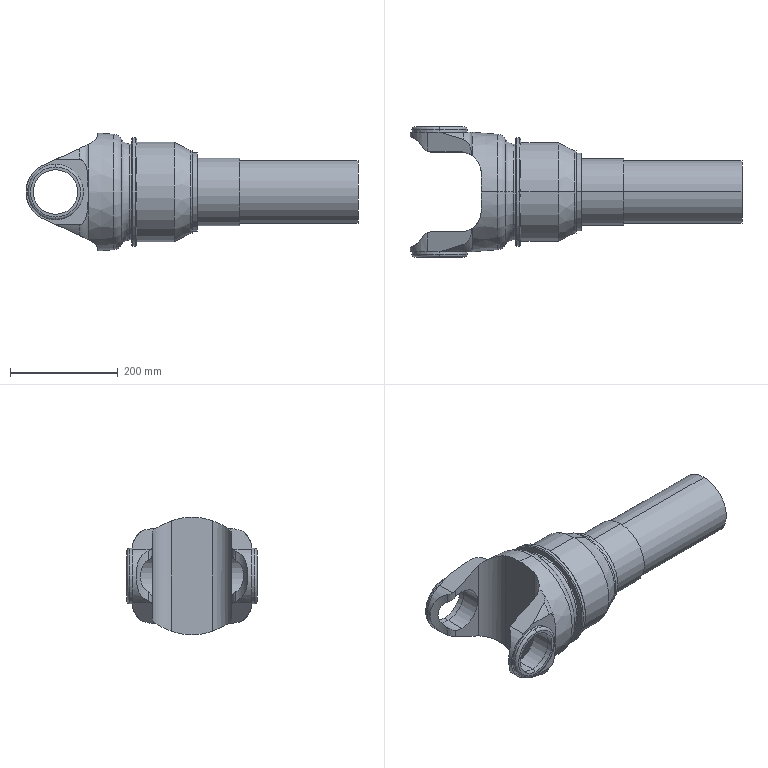Component | NX | BRAZO_PREDETERMINADO_COMO_MECANIZADA | 3 solids | 79 faces | volume 9303320 mm3 | cylinder 40 | plane 19 | torus 12 | cone 8 | commonest cylinder face diameters 83 x8 103 x4 252.513 x4 30 x4 201.927 x2 184.434 x2 153.57 x2 144.775 x2